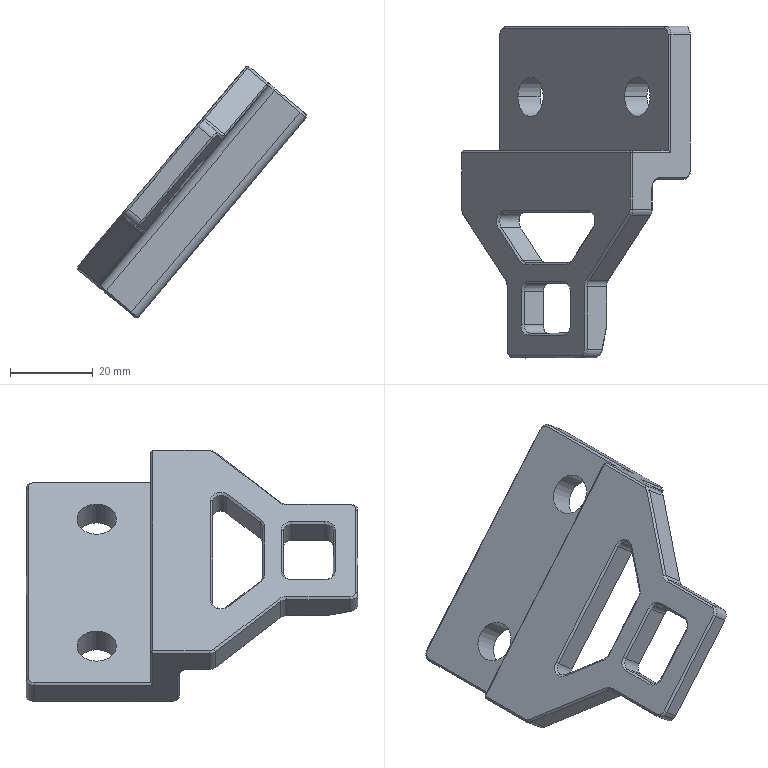Component | SolidWorks | 09GripperJawA-1 | 1 solid | 130 faces | volume 29732 mm3 | plane 68 | cone 36 | cylinder 22 | spline 4 | commonest cylinder face diameters 4 x18 9.5 x4 | material Aviation Aluminum-7075